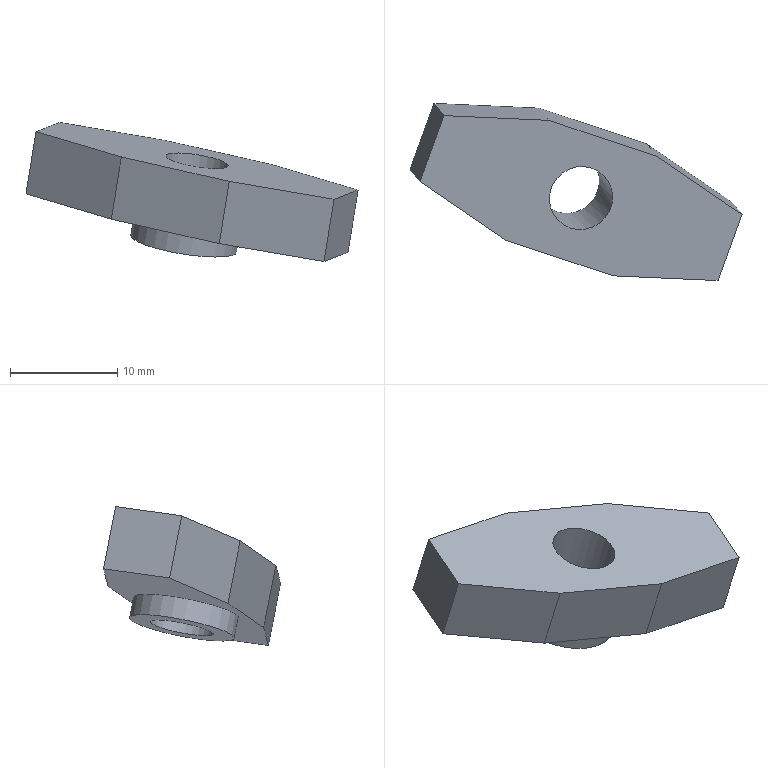Component | NX | MANUAL_NUT | 1 solid | 13 faces | box 31.02 x 16.55 x 12.98 mm | volume 1783 mm3 | plane 11 | cylinder 2 | commonest cylinder face diameters 10 x1 6 x1
STEP:
#1=CARTESIAN_POINT('',(0.,0.,0.));
#2=DIRECTION('',(0.,0.,1.));
#3=DIRECTION('',(1.,0.,0.));
#4=AXIS2_PLACEMENT_3D('',#1,#2,#3);
#5=CARTESIAN_POINT('',(-63.42,-67.809,49.572));
#6=VERTEX_POINT('',#5);
#7=CARTESIAN_POINT('',(-55.446,-73.248,47.215));
#8=VERTEX_POINT('',#7);
#9=CARTESIAN_POINT('',(-63.42,-67.809,49.572));
#10=DIRECTION('',(0.8025,-0.5474,-0.2372));
#11=VECTOR('',#10,1.);
#12=LINE('',#9,#11);
#13=CARTESIAN_POINT('',(-64.357,-66.663,43.757));
#14=DIRECTION('',(-0.5758,-0.8148,-0.06774));
#15=DIRECTION('',(-0.8025,0.5474,0.2372));
#16=AXIS2_PLACEMENT_3D('',#13,#14,#15);
#17=PLANE('',#16);
#18=CARTESIAN_POINT('',(0.,-6.));
#19=DIRECTION('',(-1.,-0.));
#20=VECTOR('',#19,1.);
#21=LINE('',#18,#20);
#22=(GEOMETRIC_REPRESENTATION_CONTEXT(2)PARAMETRIC_REPRESENTATION_CONTEXT()REPRESENTATION_CONTEXT('',''));
#23=DEFINITIONAL_REPRESENTATION('',(#21),#22);
#24=PCURVE('',#17,#23);
#25=CARTESIAN_POINT('',(-70.49,-71.734,49.938));
#26=DIRECTION('',(-0.1562,0.191,-0.9691));
#27=DIRECTION('',(-0.3378,-0.9323,-0.1293));
#28=AXIS2_PLACEMENT_3D('',#25,#26,#27);
#29=PLANE('',#28);
#30=CARTESIAN_POINT('',(-6.,-5.433));
#31=DIRECTION('',(0.2699,-0.9629));
#32=VECTOR('',#31,1.);
#33=LINE('',#30,#32);
#34=(GEOMETRIC_REPRESENTATION_CONTEXT(2)PARAMETRIC_REPRESENTATION_CONTEXT()REPRESENTATION_CONTEXT('',''));
#35=DEFINITIONAL_REPRESENTATION('',(#33),#34);
#36=PCURVE('',#29,#35);
#37=SURFACE_CURVE('',#12,(#24,#36),.PCURVE_S1.);
#38=EDGE_CURVE('',#6,#8,#37,.T.);
#39=ORIENTED_EDGE('',*,*,#38,.T.);
#40=CARTESIAN_POINT('',(-56.384,-72.102,41.4));
#41=VERTEX_POINT('',#40);
#42=CARTESIAN_POINT('',(-56.384,-72.102,41.4));
#43=DIRECTION('',(0.1562,-0.191,0.9691));
#44=VECTOR('',#43,1.);
#45=LINE('',#42,#44);
#46=CARTESIAN_POINT('',(-9.936,0.));
#47=DIRECTION('',(0.,-1.));
#48=VECTOR('',#47,1.);
#49=LINE('',#46,#48);
#50=(GEOMETRIC_REPRESENTATION_CONTEXT(2)PARAMETRIC_REPRESENTATION_CONTEXT()REPRESENTATION_CONTEXT('',''));
#51=DEFINITIONAL_REPRESENTATION('',(#49),#50);
#52=PCURVE('',#17,#51);
#53=CARTESIAN_POINT('',(-57.505,-75.196,40.971));
#54=DIRECTION('',(-0.9282,0.3072,0.2101));
#55=DIRECTION('',(-0.1562,0.191,-0.9691));
#56=AXIS2_PLACEMENT_3D('',#53,#54,#55);
#57=PLANE('',#56);
#58=CARTESIAN_POINT('',(0.,-3.318));
#59=DIRECTION('',(-1.,0.));
#60=VECTOR('',#59,1.);
#61=LINE('',#58,#60);
#62=(GEOMETRIC_REPRESENTATION_CONTEXT(2)PARAMETRIC_REPRESENTATION_CONTEXT()REPRESENTATION_CONTEXT('',''));
#63=DEFINITIONAL_REPRESENTATION('',(#61),#62);
#64=PCURVE('',#57,#63);
#65=SURFACE_CURVE('',#45,(#52,#64),.PCURVE_S1.);
#66=EDGE_CURVE('',#41,#8,#65,.T.);
#67=ORIENTED_EDGE('',*,*,#66,.F.);
#68=CARTESIAN_POINT('',(-64.357,-66.663,43.757));
#69=VERTEX_POINT('',#68);
#70=CARTESIAN_POINT('',(-64.357,-66.663,43.757));
#71=DIRECTION('',(0.8025,-0.5474,-0.2372));
#72=VECTOR('',#71,1.);
#73=LINE('',#70,#72);
#74=CARTESIAN_POINT('',(0.,0.));
#75=DIRECTION('',(-1.,-0.));
#76=VECTOR('',#75,1.);
#77=LINE('',#74,#76);
#78=(GEOMETRIC_REPRESENTATION_CONTEXT(2)PARAMETRIC_REPRESENTATION_CONTEXT()REPRESENTATION_CONTEXT('',''));
#79=DEFINITIONAL_REPRESENTATION('',(#77),#78);
#80=PCURVE('',#17,#79);
#81=CARTESIAN_POINT('',(-71.427,-70.588,44.123));
#82=DIRECTION('',(-0.1562,0.191,-0.9691));
#83=DIRECTION('',(-0.3378,-0.9323,-0.1293));
#84=AXIS2_PLACEMENT_3D('',#81,#82,#83);
#85=PLANE('',#84);
#86=CARTESIAN_POINT('',(-6.,-5.433));
#87=DIRECTION('',(0.2699,-0.9629));
#88=VECTOR('',#87,1.);
#89=LINE('',#86,#88);
#90=(GEOMETRIC_REPRESENTATION_CONTEXT(2)PARAMETRIC_REPRESENTATION_CONTEXT()REPRESENTATION_CONTEXT('',''));
#91=DEFINITIONAL_REPRESENTATION('',(#89),#90);
#92=PCURVE('',#85,#91);
#93=SURFACE_CURVE('',#73,(#80,#92),.PCURVE_S1.);
#94=EDGE_CURVE('',#69,#41,#93,.T.);
#95=ORIENTED_EDGE('',*,*,#94,.F.);
#96=CARTESIAN_POINT('',(-64.357,-66.663,43.757));
#97=DIRECTION('',(0.1562,-0.191,0.9691));
#98=VECTOR('',#97,1.);
#99=LINE('',#96,#98);
#100=CARTESIAN_POINT('',(0.,0.));
#101=DIRECTION('',(0.,-1.));
#102=VECTOR('',#101,1.);
#103=LINE('',#100,#102);
#104=(GEOMETRIC_REPRESENTATION_CONTEXT(2)PARAMETRIC_REPRESENTATION_CONTEXT()REPRESENTATION_CONTEXT('',''));
#105=DEFINITIONAL_REPRESENTATION('',(#103),#104);
#106=PCURVE('',#17,#105);
#107=CARTESIAN_POINT('',(-74.443,-63.325,46.041));
#108=DIRECTION('',(-0.3378,-0.9323,-0.1293));
#109=DIRECTION('',(-0.9282,0.3072,0.2101));
#110=AXIS2_PLACEMENT_3D('',#107,#108,#109);
#111=PLANE('',#110);
#112=CARTESIAN_POINT('',(-10.866,-0.));
#113=DIRECTION('',(0.,-1.));
#114=VECTOR('',#113,1.);
#115=LINE('',#112,#114);
#116=(GEOMETRIC_REPRESENTATION_CONTEXT(2)PARAMETRIC_REPRESENTATION_CONTEXT()REPRESENTATION_CONTEXT('',''));
#117=DEFINITIONAL_REPRESENTATION('',(#115),#116);
#118=PCURVE('',#111,#117);
#119=SURFACE_CURVE('',#99,(#106,#118),.PCURVE_S1.);
#120=EDGE_CURVE('',#69,#6,#119,.T.);
#121=ORIENTED_EDGE('',*,*,#120,.T.);
#122=EDGE_LOOP('',(#39,#67,#95,#121));
#123=FACE_BOUND('',#122,.T.);
#124=ADVANCED_FACE('',(#123),#17,.F.);
#125=CARTESIAN_POINT('',(-57.688,-79.435,46.357));
#126=VERTEX_POINT('',#125);
#127=CARTESIAN_POINT('',(-56.567,-76.341,46.786));
#128=DIRECTION('',(-0.3378,-0.9323,-0.1293));
#129=VECTOR('',#128,1.);
#130=LINE('',#127,#129);
#131=CARTESIAN_POINT('',(-6.,0.));
#132=DIRECTION('',(-0.,1.));
#133=VECTOR('',#132,1.);
#134=LINE('',#131,#133);
#135=(GEOMETRIC_REPRESENTATION_CONTEXT(2)PARAMETRIC_REPRESENTATION_CONTEXT()REPRESENTATION_CONTEXT('',''));
#136=DEFINITIONAL_REPRESENTATION('',(#134),#135);
#137=PCURVE('',#57,#136);
#138=CARTESIAN_POINT('',(0.,-15.));
#139=DIRECTION('',(1.,-0.));
#140=VECTOR('',#139,1.);
#141=LINE('',#138,#140);
#142=(GEOMETRIC_REPRESENTATION_CONTEXT(2)PARAMETRIC_REPRESENTATION_CONTEXT()REPRESENTATION_CONTEXT('',''));
#143=DEFINITIONAL_REPRESENTATION('',(#141),#142);
#144=PCURVE('',#29,#143);
#145=SURFACE_CURVE('',#130,(#137,#144),.PCURVE_S1.);
#146=EDGE_CURVE('',#8,#126,#145,.T.);
#147=ORIENTED_EDGE('',*,*,#146,.T.);
#148=CARTESIAN_POINT('',(-58.625,-78.289,40.542));
#149=VERTEX_POINT('',#148);
#150=CARTESIAN_POINT('',(-58.625,-78.289,40.542));
#151=DIRECTION('',(0.1562,-0.191,0.9691));
#152=VECTOR('',#151,1.);
#153=LINE('',#150,#152);
#154=CARTESIAN_POINT('',(-0.,3.318));
#155=DIRECTION('',(-1.,0.));
#156=VECTOR('',#155,1.);
#157=LINE('',#154,#156);
#158=(GEOMETRIC_REPRESENTATION_CONTEXT(2)PARAMETRIC_REPRESENTATION_CONTEXT()REPRESENTATION_CONTEXT('',''));
#159=DEFINITIONAL_REPRESENTATION('',(#157),#158);
#160=PCURVE('',#57,#159);
#161=CARTESIAN_POINT('',(-58.625,-78.289,40.542));
#162=DIRECTION('',(0.07475,0.9806,0.1812));
#163=DIRECTION('',(0.9849,-0.04414,-0.1674));
#164=AXIS2_PLACEMENT_3D('',#161,#162,#163);
#165=PLANE('',#164);
#166=CARTESIAN_POINT('',(0.,0.));
#167=DIRECTION('',(-0.,-1.));
#168=VECTOR('',#167,1.);
#169=LINE('',#166,#168);
#170=(GEOMETRIC_REPRESENTATION_CONTEXT(2)PARAMETRIC_REPRESENTATION_CONTEXT()REPRESENTATION_CONTEXT('',''));
#171=DEFINITIONAL_REPRESENTATION('',(#169),#170);
#172=PCURVE('',#165,#171);
#173=SURFACE_CURVE('',#153,(#160,#172),.PCURVE_S1.);
#174=EDGE_CURVE('',#149,#126,#173,.T.);
#175=ORIENTED_EDGE('',*,*,#174,.F.);
#176=CARTESIAN_POINT('',(-56.384,-72.102,41.4));
#177=DIRECTION('',(-0.3378,-0.9323,-0.1293));
#178=VECTOR('',#177,1.);
#179=LINE('',#176,#178);
#180=CARTESIAN_POINT('',(0.,-3.318));
#181=DIRECTION('',(-0.,1.));
#182=VECTOR('',#181,1.);
#183=LINE('',#180,#182);
#184=(GEOMETRIC_REPRESENTATION_CONTEXT(2)PARAMETRIC_REPRESENTATION_CONTEXT()REPRESENTATION_CONTEXT('',''));
#185=DEFINITIONAL_REPRESENTATION('',(#183),#184);
#186=PCURVE('',#57,#185);
#187=CARTESIAN_POINT('',(-3.318,-15.));
#188=DIRECTION('',(1.,-0.));
#189=VECTOR('',#188,1.);
#190=LINE('',#187,#189);
#191=(GEOMETRIC_REPRESENTATION_CONTEXT(2)PARAMETRIC_REPRESENTATION_CONTEXT()REPRESENTATION_CONTEXT('',''));
#192=DEFINITIONAL_REPRESENTATION('',(#190),#191);
#193=PCURVE('',#85,#192);
#194=SURFACE_CURVE('',#179,(#186,#193),.PCURVE_S1.);
#195=EDGE_CURVE('',#41,#149,#194,.T.);
#196=ORIENTED_EDGE('',*,*,#195,.F.);
#197=ORIENTED_EDGE('',*,*,#66,.T.);
#198=EDGE_LOOP('',(#147,#175,#196,#197));
#199=FACE_BOUND('',#198,.T.);
#200=ADVANCED_FACE('',(#199),#57,.F.);
#201=CARTESIAN_POINT('',(-67.474,-78.996,48.021));
#202=VERTEX_POINT('',#201);
#203=CARTESIAN_POINT('',(-57.688,-79.435,46.357));
#204=DIRECTION('',(-0.9849,0.04414,0.1674));
#205=VECTOR('',#204,1.);
#206=LINE('',#203,#205);
#207=CARTESIAN_POINT('',(0.,-6.));
#208=DIRECTION('',(-1.,0.));
#209=VECTOR('',#208,1.);
#210=LINE('',#207,#209);
#211=(GEOMETRIC_REPRESENTATION_CONTEXT(2)PARAMETRIC_REPRESENTATION_CONTEXT()REPRESENTATION_CONTEXT('',''));
#212=DEFINITIONAL_REPRESENTATION('',(#210),#211);
#213=PCURVE('',#165,#212);
#214=CARTESIAN_POINT('',(3.318,-15.));
#215=DIRECTION('',(0.2699,0.9629));
#216=VECTOR('',#215,1.);
#217=LINE('',#214,#216);
#218=(GEOMETRIC_REPRESENTATION_CONTEXT(2)PARAMETRIC_REPRESENTATION_CONTEXT()REPRESENTATION_CONTEXT('',''));
#219=DEFINITIONAL_REPRESENTATION('',(#217),#218);
#220=PCURVE('',#29,#219);
#221=SURFACE_CURVE('',#206,(#213,#220),.PCURVE_S1.);
#222=EDGE_CURVE('',#126,#202,#221,.T.);
#223=ORIENTED_EDGE('',*,*,#222,.T.);
#224=CARTESIAN_POINT('',(-68.411,-77.851,42.206));
#225=VERTEX_POINT('',#224);
#226=CARTESIAN_POINT('',(-68.411,-77.851,42.206));
#227=DIRECTION('',(0.1562,-0.191,0.9691));
#228=VECTOR('',#227,1.);
#229=LINE('',#226,#228);
#230=CARTESIAN_POINT('',(-9.936,0.));
#231=DIRECTION('',(-0.,-1.));
#232=VECTOR('',#231,1.);
#233=LINE('',#230,#232);
#234=(GEOMETRIC_REPRESENTATION_CONTEXT(2)PARAMETRIC_REPRESENTATION_CONTEXT()REPRESENTATION_CONTEXT('',''));
#235=DEFINITIONAL_REPRESENTATION('',(#233),#234);
#236=PCURVE('',#165,#235);
#237=CARTESIAN_POINT('',(-73.454,-76.182,43.348));
#238=DIRECTION('',(0.3378,0.9323,0.1293));
#239=DIRECTION('',(0.9282,-0.3072,-0.2101));
#240=AXIS2_PLACEMENT_3D('',#237,#238,#239);
#241=PLANE('',#240);
#242=CARTESIAN_POINT('',(5.433,-0.));
#243=DIRECTION('',(0.,-1.));
#244=VECTOR('',#243,1.);
#245=LINE('',#242,#244);
#246=(GEOMETRIC_REPRESENTATION_CONTEXT(2)PARAMETRIC_REPRESENTATION_CONTEXT()REPRESENTATION_CONTEXT('',''));
#247=DEFINITIONAL_REPRESENTATION('',(#245),#246);
#248=PCURVE('',#241,#247);
#249=SURFACE_CURVE('',#229,(#236,#248),.PCURVE_S1.);
#250=EDGE_CURVE('',#225,#202,#249,.T.);
#251=ORIENTED_EDGE('',*,*,#250,.F.);
#252=CARTESIAN_POINT('',(-58.625,-78.289,40.542));
#253=DIRECTION('',(-0.9849,0.04414,0.1674));
#254=VECTOR('',#253,1.);
#255=LINE('',#252,#254);
#256=CARTESIAN_POINT('',(0.,0.));
#257=DIRECTION('',(-1.,0.));
#258=VECTOR('',#257,1.);
#259=LINE('',#256,#258);
#260=(GEOMETRIC_REPRESENTATION_CONTEXT(2)PARAMETRIC_REPRESENTATION_CONTEXT()REPRESENTATION_CONTEXT('',''));
#261=DEFINITIONAL_REPRESENTATION('',(#259),#260);
#262=PCURVE('',#165,#261);
#263=CARTESIAN_POINT('',(3.318,-15.));
#264=DIRECTION('',(0.2699,0.9629));
#265=VECTOR('',#264,1.);
#266=LINE('',#263,#265);
#267=(GEOMETRIC_REPRESENTATION_CONTEXT(2)PARAMETRIC_REPRESENTATION_CONTEXT()REPRESENTATION_CONTEXT('',''));
#268=DEFINITIONAL_REPRESENTATION('',(#266),#267);
#269=PCURVE('',#85,#268);
#270=SURFACE_CURVE('',#255,(#262,#269),.PCURVE_S1.);
#271=EDGE_CURVE('',#149,#225,#270,.T.);
#272=ORIENTED_EDGE('',*,*,#271,.F.);
#273=ORIENTED_EDGE('',*,*,#174,.T.);
#274=EDGE_LOOP('',(#223,#251,#272,#273));
#275=FACE_BOUND('',#274,.T.);
#276=ADVANCED_FACE('',(#275),#165,.F.);
#277=CARTESIAN_POINT('',(-77.56,-75.658,50.304));
#278=VERTEX_POINT('',#277);
#279=CARTESIAN_POINT('',(-72.517,-77.327,49.162));
#280=DIRECTION('',(-0.9282,0.3072,0.2101));
#281=VECTOR('',#280,1.);
#282=LINE('',#279,#281);
#283=CARTESIAN_POINT('',(0.,-6.));
#284=DIRECTION('',(-1.,0.));
#285=VECTOR('',#284,1.);
#286=LINE('',#283,#285);
#287=(GEOMETRIC_REPRESENTATION_CONTEXT(2)PARAMETRIC_REPRESENTATION_CONTEXT()REPRESENTATION_CONTEXT('',''));
#288=DEFINITIONAL_REPRESENTATION('',(#286),#287);
#289=PCURVE('',#241,#288);
#290=CARTESIAN_POINT('',(6.,-0.));
#291=DIRECTION('',(0.,1.));
#292=VECTOR('',#291,1.);
#293=LINE('',#290,#292);
#294=(GEOMETRIC_REPRESENTATION_CONTEXT(2)PARAMETRIC_REPRESENTATION_CONTEXT()REPRESENTATION_CONTEXT('',''));
#295=DEFINITIONAL_REPRESENTATION('',(#293),#294);
#296=PCURVE('',#29,#295);
#297=SURFACE_CURVE('',#282,(#289,#296),.PCURVE_S1.);
#298=EDGE_CURVE('',#202,#278,#297,.T.);
#299=ORIENTED_EDGE('',*,*,#298,.T.);
#300=CARTESIAN_POINT('',(-78.497,-74.513,44.489));
#301=VERTEX_POINT('',#300);
#302=CARTESIAN_POINT('',(-78.497,-74.513,44.489));
#303=DIRECTION('',(0.1562,-0.191,0.9691));
#304=VECTOR('',#303,1.);
#305=LINE('',#302,#304);
#306=CARTESIAN_POINT('',(-5.433,-0.));
#307=DIRECTION('',(0.,-1.));
#308=VECTOR('',#307,1.);
#309=LINE('',#306,#308);
#310=(GEOMETRIC_REPRESENTATION_CONTEXT(2)PARAMETRIC_REPRESENTATION_CONTEXT()REPRESENTATION_CONTEXT('',''));
#311=DEFINITIONAL_REPRESENTATION('',(#309),#310);
#312=PCURVE('',#241,#311);
#313=CARTESIAN_POINT('',(-78.497,-74.513,44.489));
#314=DIRECTION('',(0.5758,0.8148,0.06774));
#315=DIRECTION('',(0.8025,-0.5474,-0.2372));
#316=AXIS2_PLACEMENT_3D('',#313,#314,#315);
#317=PLANE('',#316);
#318=CARTESIAN_POINT('',(0.,0.));
#319=DIRECTION('',(-0.,-1.));
#320=VECTOR('',#319,1.);
#321=LINE('',#318,#320);
#322=(GEOMETRIC_REPRESENTATION_CONTEXT(2)PARAMETRIC_REPRESENTATION_CONTEXT()REPRESENTATION_CONTEXT('',''));
#323=DEFINITIONAL_REPRESENTATION('',(#321),#322);
#324=PCURVE('',#317,#323);
#325=SURFACE_CURVE('',#305,(#312,#324),.PCURVE_S1.);
#326=EDGE_CURVE('',#301,#278,#325,.T.);
#327=ORIENTED_EDGE('',*,*,#326,.F.);
#328=CARTESIAN_POINT('',(-68.411,-77.851,42.206));
#329=DIRECTION('',(-0.9282,0.3072,0.2101));
#330=VECTOR('',#329,1.);
#331=LINE('',#328,#330);
#332=CARTESIAN_POINT('',(5.433,-0.));
#333=DIRECTION('',(-1.,-0.));
#334=VECTOR('',#333,1.);
#335=LINE('',#332,#334);
#336=(GEOMETRIC_REPRESENTATION_CONTEXT(2)PARAMETRIC_REPRESENTATION_CONTEXT()REPRESENTATION_CONTEXT('',''));
#337=DEFINITIONAL_REPRESENTATION('',(#335),#336);
#338=PCURVE('',#241,#337);
#339=CARTESIAN_POINT('',(6.,-5.433));
#340=DIRECTION('',(-0.,1.));
#341=VECTOR('',#340,1.);
#342=LINE('',#339,#341);
#343=(GEOMETRIC_REPRESENTATION_CONTEXT(2)PARAMETRIC_REPRESENTATION_CONTEXT()REPRESENTATION_CONTEXT('',''));
#344=DEFINITIONAL_REPRESENTATION('',(#342),#343);
#345=PCURVE('',#85,#344);
#346=SURFACE_CURVE('',#331,(#338,#345),.PCURVE_S1.);
#347=EDGE_CURVE('',#225,#301,#346,.T.);
#348=ORIENTED_EDGE('',*,*,#347,.F.);
#349=ORIENTED_EDGE('',*,*,#250,.T.);
#350=EDGE_LOOP('',(#299,#327,#348,#349));
#351=FACE_BOUND('',#350,.T.);
#352=ADVANCED_FACE('',(#351),#241,.F.);
#353=CARTESIAN_POINT('',(-85.533,-70.219,52.661));
#354=VERTEX_POINT('',#353);
#355=CARTESIAN_POINT('',(-77.56,-75.658,50.304));
#356=DIRECTION('',(-0.8025,0.5474,0.2372));
#357=VECTOR('',#356,1.);
#358=LINE('',#355,#357);
#359=CARTESIAN_POINT('',(0.,-6.));
#360=DIRECTION('',(-1.,0.));
#361=VECTOR('',#360,1.);
#362=LINE('',#359,#361);
#363=(GEOMETRIC_REPRESENTATION_CONTEXT(2)PARAMETRIC_REPRESENTATION_CONTEXT()REPRESENTATION_CONTEXT('',''));
#364=DEFINITIONAL_REPRESENTATION('',(#362),#363);
#365=PCURVE('',#317,#364);
#366=CARTESIAN_POINT('',(6.,5.433));
#367=DIRECTION('',(-0.2699,0.9629));
#368=VECTOR('',#367,1.);
#369=LINE('',#366,#368);
#370=(GEOMETRIC_REPRESENTATION_CONTEXT(2)PARAMETRIC_REPRESENTATION_CONTEXT()REPRESENTATION_CONTEXT('',''));
#371=DEFINITIONAL_REPRESENTATION('',(#369),#370);
#372=PCURVE('',#29,#371);
#373=SURFACE_CURVE('',#358,(#365,#372),.PCURVE_S1.);
#374=EDGE_CURVE('',#278,#354,#373,.T.);
#375=ORIENTED_EDGE('',*,*,#374,.T.);
#376=CARTESIAN_POINT('',(-86.47,-69.073,46.846));
#377=VERTEX_POINT('',#376);
#378=CARTESIAN_POINT('',(-86.47,-69.073,46.846));
#379=DIRECTION('',(0.1562,-0.191,0.9691));
#380=VECTOR('',#379,1.);
#381=LINE('',#378,#380);
#382=CARTESIAN_POINT('',(-9.936,-0.));
#383=DIRECTION('',(-0.,-1.));
#384=VECTOR('',#383,1.);
#385=LINE('',#382,#384);
#386=(GEOMETRIC_REPRESENTATION_CONTEXT(2)PARAMETRIC_REPRESENTATION_CONTEXT()REPRESENTATION_CONTEXT('',''));
#387=DEFINITIONAL_REPRESENTATION('',(#385),#386);
#388=PCURVE('',#317,#387);
#389=CARTESIAN_POINT('',(-85.349,-65.98,47.275));
#390=DIRECTION('',(0.9282,-0.3072,-0.2101));
#391=DIRECTION('',(0.1562,-0.191,0.9691));
#392=AXIS2_PLACEMENT_3D('',#389,#390,#391);
#393=PLANE('',#392);
#394=CARTESIAN_POINT('',(0.,3.318));
#395=DIRECTION('',(1.,0.));
#396=VECTOR('',#395,1.);
#397=LINE('',#394,#396);
#398=(GEOMETRIC_REPRESENTATION_CONTEXT(2)PARAMETRIC_REPRESENTATION_CONTEXT()REPRESENTATION_CONTEXT('',''));
#399=DEFINITIONAL_REPRESENTATION('',(#397),#398);
#400=PCURVE('',#393,#399);
#401=SURFACE_CURVE('',#381,(#388,#400),.PCURVE_S1.);
#402=EDGE_CURVE('',#377,#354,#401,.T.);
#403=ORIENTED_EDGE('',*,*,#402,.F.);
#404=CARTESIAN_POINT('',(-78.497,-74.513,44.489));
#405=DIRECTION('',(-0.8025,0.5474,0.2372));
#406=VECTOR('',#405,1.);
#407=LINE('',#404,#406);
#408=CARTESIAN_POINT('',(0.,0.));
#409=DIRECTION('',(-1.,0.));
#410=VECTOR('',#409,1.);
#411=LINE('',#408,#410);
#412=(GEOMETRIC_REPRESENTATION_CONTEXT(2)PARAMETRIC_REPRESENTATION_CONTEXT()REPRESENTATION_CONTEXT('',''));
#413=DEFINITIONAL_REPRESENTATION('',(#411),#412);
#414=PCURVE('',#317,#413);
#415=CARTESIAN_POINT('',(6.,5.433));
#416=DIRECTION('',(-0.2699,0.9629));
#417=VECTOR('',#416,1.);
#418=LINE('',#415,#417);
#419=(GEOMETRIC_REPRESENTATION_CONTEXT(2)PARAMETRIC_REPRESENTATION_CONTEXT()REPRESENTATION_CONTEXT('',''));
#420=DEFINITIONAL_REPRESENTATION('',(#418),#419);
#421=PCURVE('',#85,#420);
#422=SURFACE_CURVE('',#407,(#414,#421),.PCURVE_S1.);
#423=EDGE_CURVE('',#301,#377,#422,.T.);
#424=ORIENTED_EDGE('',*,*,#423,.F.);
#425=ORIENTED_EDGE('',*,*,#326,.T.);
#426=EDGE_LOOP('',(#375,#403,#424,#425));
#427=FACE_BOUND('',#426,.T.);
#428=ADVANCED_FACE('',(#427),#317,.F.);
#429=CARTESIAN_POINT('',(-83.291,-64.032,53.519));
#430=VERTEX_POINT('',#429);
#431=CARTESIAN_POINT('',(-84.412,-67.126,53.09));
#432=DIRECTION('',(0.3378,0.9323,0.1293));
#433=VECTOR('',#432,1.);
#434=LINE('',#431,#433);
#435=CARTESIAN_POINT('',(6.,-0.));
#436=DIRECTION('',(-0.,-1.));
#437=VECTOR('',#436,1.);
#438=LINE('',#435,#437);
#439=(GEOMETRIC_REPRESENTATION_CONTEXT(2)PARAMETRIC_REPRESENTATION_CONTEXT()REPRESENTATION_CONTEXT('',''));
#440=DEFINITIONAL_REPRESENTATION('',(#438),#439);
#441=PCURVE('',#393,#440);
#442=CARTESIAN_POINT('',(-0.,15.));
#443=DIRECTION('',(-1.,0.));
#444=VECTOR('',#443,1.);
#445=LINE('',#442,#444);
#446=(GEOMETRIC_REPRESENTATION_CONTEXT(2)PARAMETRIC_REPRESENTATION_CONTEXT()REPRESENTATION_CONTEXT('',''));
#447=DEFINITIONAL_REPRESENTATION('',(#445),#446);
#448=PCURVE('',#29,#447);
#449=SURFACE_CURVE('',#434,(#441,#448),.PCURVE_S1.);
#450=EDGE_CURVE('',#354,#430,#449,.T.);
#451=ORIENTED_EDGE('',*,*,#450,.T.);
#452=CARTESIAN_POINT('',(-84.228,-62.886,47.704));
#453=VERTEX_POINT('',#452);
#454=CARTESIAN_POINT('',(-84.228,-62.886,47.704));
#455=DIRECTION('',(0.1562,-0.191,0.9691));
#456=VECTOR('',#455,1.);
#457=LINE('',#454,#456);
#458=CARTESIAN_POINT('',(0.,-3.318));
#459=DIRECTION('',(1.,0.));
#460=VECTOR('',#459,1.);
#461=LINE('',#458,#460);
#462=(GEOMETRIC_REPRESENTATION_CONTEXT(2)PARAMETRIC_REPRESENTATION_CONTEXT()REPRESENTATION_CONTEXT('',''));
#463=DEFINITIONAL_REPRESENTATION('',(#461),#462);
#464=PCURVE('',#393,#463);
#465=CARTESIAN_POINT('',(-84.228,-62.886,47.704));
#466=DIRECTION('',(-0.07475,-0.9806,-0.1812));
#467=DIRECTION('',(-0.9849,0.04414,0.1674));
#468=AXIS2_PLACEMENT_3D('',#465,#466,#467);
#469=PLANE('',#468);
#470=CARTESIAN_POINT('',(0.,0.));
#471=DIRECTION('',(0.,-1.));
#472=VECTOR('',#471,1.);
#473=LINE('',#470,#472);
#474=(GEOMETRIC_REPRESENTATION_CONTEXT(2)PARAMETRIC_REPRESENTATION_CONTEXT()REPRESENTATION_CONTEXT('',''));
#475=DEFINITIONAL_REPRESENTATION('',(#473),#474);
#476=PCURVE('',#469,#475);
#477=SURFACE_CURVE('',#457,(#464,#476),.PCURVE_S1.);
#478=EDGE_CURVE('',#453,#430,#477,.T.);
#479=ORIENTED_EDGE('',*,*,#478,.F.);
#480=CARTESIAN_POINT('',(-86.47,-69.073,46.846));
#481=DIRECTION('',(0.3378,0.9323,0.1293));
#482=VECTOR('',#481,1.);
#483=LINE('',#480,#482);
#484=CARTESIAN_POINT('',(0.,3.318));
#485=DIRECTION('',(-0.,-1.));
#486=VECTOR('',#485,1.);
#487=LINE('',#484,#486);
#488=(GEOMETRIC_REPRESENTATION_CONTEXT(2)PARAMETRIC_REPRESENTATION_CONTEXT()REPRESENTATION_CONTEXT('',''));
#489=DEFINITIONAL_REPRESENTATION('',(#487),#488);
#490=PCURVE('',#393,#489);
#491=CARTESIAN_POINT('',(3.318,15.));
#492=DIRECTION('',(-1.,0.));
#493=VECTOR('',#492,1.);
#494=LINE('',#491,#493);
#495=(GEOMETRIC_REPRESENTATION_CONTEXT(2)PARAMETRIC_REPRESENTATION_CONTEXT()REPRESENTATION_CONTEXT('',''));
#496=DEFINITIONAL_REPRESENTATION('',(#494),#495);
#497=PCURVE('',#85,#496);
#498=SURFACE_CURVE('',#483,(#490,#497),.PCURVE_S1.);
#499=EDGE_CURVE('',#377,#453,#498,.T.);
#500=ORIENTED_EDGE('',*,*,#499,.F.);
#501=ORIENTED_EDGE('',*,*,#402,.T.);
#502=EDGE_LOOP('',(#451,#479,#500,#501));
#503=FACE_BOUND('',#502,.T.);
#504=ADVANCED_FACE('',(#503),#393,.F.);
#505=CARTESIAN_POINT('',(-73.506,-64.471,51.855));
#506=VERTEX_POINT('',#505);
#507=CARTESIAN_POINT('',(-83.291,-64.032,53.519));
#508=DIRECTION('',(0.9849,-0.04414,-0.1674));
#509=VECTOR('',#508,1.);
#510=LINE('',#507,#509);
#511=CARTESIAN_POINT('',(-0.,-6.));
#512=DIRECTION('',(-1.,-0.));
#513=VECTOR('',#512,1.);
#514=LINE('',#511,#513);
#515=(GEOMETRIC_REPRESENTATION_CONTEXT(2)PARAMETRIC_REPRESENTATION_CONTEXT()REPRESENTATION_CONTEXT('',''));
#516=DEFINITIONAL_REPRESENTATION('',(#514),#515);
#517=PCURVE('',#469,#516);
#518=CARTESIAN_POINT('',(-3.318,15.));
#519=DIRECTION('',(-0.2699,-0.9629));
#520=VECTOR('',#519,1.);
#521=LINE('',#518,#520);
#522=(GEOMETRIC_REPRESENTATION_CONTEXT(2)PARAMETRIC_REPRESENTATION_CONTEXT()REPRESENTATION_CONTEXT('',''));
#523=DEFINITIONAL_REPRESENTATION('',(#521),#522);
#524=PCURVE('',#29,#523);
#525=SURFACE_CURVE('',#510,(#517,#524),.PCURVE_S1.);
#526=EDGE_CURVE('',#430,#506,#525,.T.);
#527=ORIENTED_EDGE('',*,*,#526,.T.);
#528=CARTESIAN_POINT('',(-74.443,-63.325,46.041));
#529=VERTEX_POINT('',#528);
#530=CARTESIAN_POINT('',(-74.443,-63.325,46.041));
#531=DIRECTION('',(0.1562,-0.191,0.9691));
#532=VECTOR('',#531,1.);
#533=LINE('',#530,#532);
#534=CARTESIAN_POINT('',(-9.936,0.));
#535=DIRECTION('',(0.,-1.));
#536=VECTOR('',#535,1.);
#537=LINE('',#534,#536);
#538=(GEOMETRIC_REPRESENTATION_CONTEXT(2)PARAMETRIC_REPRESENTATION_CONTEXT()REPRESENTATION_CONTEXT('',''));
#539=DEFINITIONAL_REPRESENTATION('',(#537),#538);
#540=PCURVE('',#469,#539);
#541=CARTESIAN_POINT('',(0.,0.));
#542=DIRECTION('',(0.,-1.));
#543=VECTOR('',#542,1.);
#544=LINE('',#541,#543);
#545=(GEOMETRIC_REPRESENTATION_CONTEXT(2)PARAMETRIC_REPRESENTATION_CONTEXT()REPRESENTATION_CONTEXT('',''));
#546=DEFINITIONAL_REPRESENTATION('',(#544),#545);
#547=PCURVE('',#111,#546);
#548=SURFACE_CURVE('',#533,(#540,#547),.PCURVE_S1.);
#549=EDGE_CURVE('',#529,#506,#548,.T.);
#550=ORIENTED_EDGE('',*,*,#549,.F.);
#551=CARTESIAN_POINT('',(-84.228,-62.886,47.704));
#552=DIRECTION('',(0.9849,-0.04414,-0.1674));
#553=VECTOR('',#552,1.);
#554=LINE('',#551,#553);
#555=CARTESIAN_POINT('',(0.,0.));
#556=DIRECTION('',(-1.,-0.));
#557=VECTOR('',#556,1.);
#558=LINE('',#555,#557);
#559=(GEOMETRIC_REPRESENTATION_CONTEXT(2)PARAMETRIC_REPRESENTATION_CONTEXT()REPRESENTATION_CONTEXT('',''));
#560=DEFINITIONAL_REPRESENTATION('',(#558),#559);
#561=PCURVE('',#469,#560);
#562=CARTESIAN_POINT('',(-3.318,15.));
#563=DIRECTION('',(-0.2699,-0.9629));
#564=VECTOR('',#563,1.);
#565=LINE('',#562,#564);
#566=(GEOMETRIC_REPRESENTATION_CONTEXT(2)PARAMETRIC_REPRESENTATION_CONTEXT()REPRESENTATION_CONTEXT('',''));
#567=DEFINITIONAL_REPRESENTATION('',(#565),#566);
#568=PCURVE('',#85,#567);
#569=SURFACE_CURVE('',#554,(#561,#568),.PCURVE_S1.);
#570=EDGE_CURVE('',#453,#529,#569,.T.);
#571=ORIENTED_EDGE('',*,*,#570,.F.);
#572=ORIENTED_EDGE('',*,*,#478,.T.);
#573=EDGE_LOOP('',(#527,#550,#571,#572));
#574=FACE_BOUND('',#573,.T.);
#575=ADVANCED_FACE('',(#574),#469,.F.);
#576=CARTESIAN_POINT('',(-73.506,-64.471,51.855));
#577=DIRECTION('',(0.9282,-0.3072,-0.2101));
#578=VECTOR('',#577,1.);
#579=LINE('',#576,#578);
#580=CARTESIAN_POINT('',(0.,-6.));
#581=DIRECTION('',(-1.,0.));
#582=VECTOR('',#581,1.);
#583=LINE('',#580,#582);
#584=(GEOMETRIC_REPRESENTATION_CONTEXT(2)PARAMETRIC_REPRESENTATION_CONTEXT()REPRESENTATION_CONTEXT('',''));
#585=DEFINITIONAL_REPRESENTATION('',(#583),#584);
#586=PCURVE('',#111,#585);
#587=CARTESIAN_POINT('',(-6.,5.433));
#588=DIRECTION('',(0.,-1.));
#589=VECTOR('',#588,1.);
#590=LINE('',#587,#589);
#591=(GEOMETRIC_REPRESENTATION_CONTEXT(2)PARAMETRIC_REPRESENTATION_CONTEXT()REPRESENTATION_CONTEXT('',''));
#592=DEFINITIONAL_REPRESENTATION('',(#590),#591);
#593=PCURVE('',#29,#592);
#594=SURFACE_CURVE('',#579,(#586,#593),.PCURVE_S1.);
#595=EDGE_CURVE('',#506,#6,#594,.T.);
#596=ORIENTED_EDGE('',*,*,#595,.T.);
#597=ORIENTED_EDGE('',*,*,#120,.F.);
#598=CARTESIAN_POINT('',(-69.4,-64.994,44.899));
#599=DIRECTION('',(0.9282,-0.3072,-0.2101));
#600=VECTOR('',#599,1.);
#601=LINE('',#598,#600);
#602=CARTESIAN_POINT('',(-5.433,0.));
#603=DIRECTION('',(-1.,-0.));
#604=VECTOR('',#603,1.);
#605=LINE('',#602,#604);
#606=(GEOMETRIC_REPRESENTATION_CONTEXT(2)PARAMETRIC_REPRESENTATION_CONTEXT()REPRESENTATION_CONTEXT('',''));
#607=DEFINITIONAL_REPRESENTATION('',(#605),#606);
#608=PCURVE('',#111,#607);
#609=CARTESIAN_POINT('',(-6.,-0.));
#610=DIRECTION('',(-0.,-1.));
#611=VECTOR('',#610,1.);
#612=LINE('',#609,#611);
#613=(GEOMETRIC_REPRESENTATION_CONTEXT(2)PARAMETRIC_REPRESENTATION_CONTEXT()REPRESENTATION_CONTEXT('',''));
#614=DEFINITIONAL_REPRESENTATION('',(#612),#613);
#615=PCURVE('',#85,#614);
#616=SURFACE_CURVE('',#601,(#608,#615),.PCURVE_S1.);
#617=EDGE_CURVE('',#529,#69,#616,.T.);
#618=ORIENTED_EDGE('',*,*,#617,.F.);
#619=ORIENTED_EDGE('',*,*,#549,.T.);
#620=EDGE_LOOP('',(#596,#597,#618,#619));
#621=FACE_BOUND('',#620,.T.);
#622=ADVANCED_FACE('',(#621),#111,.F.);
#623=CARTESIAN_POINT('',(-73.116,-75.249,43.477));
#624=VERTEX_POINT('',#623);
#625=CARTESIAN_POINT('',(-71.427,-70.588,44.123));
#626=DIRECTION('',(-0.1562,0.191,-0.9691));
#627=DIRECTION('',(-0.3378,-0.9323,-0.1293));
#628=AXIS2_PLACEMENT_3D('',#625,#626,#627);
#629=CIRCLE('',#628,5.);
#630=CARTESIAN_POINT('',(0.,0.));
#631=DIRECTION('',(1.,0.));
#632=AXIS2_PLACEMENT_2D('',#630,#631);
#633=CIRCLE('',#632,5.);
#634=(GEOMETRIC_REPRESENTATION_CONTEXT(2)PARAMETRIC_REPRESENTATION_CONTEXT()REPRESENTATION_CONTEXT('',''));
#635=DEFINITIONAL_REPRESENTATION('',(#633),#634);
#636=PCURVE('',#85,#635);
#637=CARTESIAN_POINT('',(-71.739,-70.206,42.185));
#638=DIRECTION('',(0.1562,-0.191,0.9691));
#639=DIRECTION('',(0.3378,0.9323,0.1293));
#640=AXIS2_PLACEMENT_3D('',#637,#638,#639);
#641=CYLINDRICAL_SURFACE('',#640,5.);
#642=CARTESIAN_POINT('',(9.425,2.));
#643=DIRECTION('',(-1.,0.));
#644=VECTOR('',#643,1.);
#645=LINE('',#642,#644);
#646=(GEOMETRIC_REPRESENTATION_CONTEXT(2)PARAMETRIC_REPRESENTATION_CONTEXT()REPRESENTATION_CONTEXT('',''));
#647=DEFINITIONAL_REPRESENTATION('',(#645),#646);
#648=PCURVE('',#641,#647);
#649=SURFACE_CURVE('',#629,(#636,#648),.PCURVE_S1.);
#650=EDGE_CURVE('',#624,#624,#649,.T.);
#651=ORIENTED_EDGE('',*,*,#650,.F.);
#652=EDGE_LOOP('',(#651));
#653=FACE_BOUND('',#652,.T.);
#654=ORIENTED_EDGE('',*,*,#617,.T.);
#655=ORIENTED_EDGE('',*,*,#94,.T.);
#656=ORIENTED_EDGE('',*,*,#195,.T.);
#657=ORIENTED_EDGE('',*,*,#271,.T.);
#658=ORIENTED_EDGE('',*,*,#347,.T.);
#659=ORIENTED_EDGE('',*,*,#423,.T.);
#660=ORIENTED_EDGE('',*,*,#499,.T.);
#661=ORIENTED_EDGE('',*,*,#570,.T.);
#662=EDGE_LOOP('',(#654,#655,#656,#657,#658,#659,#660,#661));
#663=FACE_BOUND('',#662,.T.);
#664=ADVANCED_FACE('',(#653,#663),#85,.T.);
#665=CARTESIAN_POINT('',(-71.503,-74.53,49.55));
#666=VERTEX_POINT('',#665);
#667=CARTESIAN_POINT('',(-70.49,-71.734,49.938));
#668=DIRECTION('',(-0.1562,0.191,-0.9691));
#669=DIRECTION('',(-0.3378,-0.9323,-0.1293));
#670=AXIS2_PLACEMENT_3D('',#667,#668,#669);
#671=CIRCLE('',#670,3.);
#672=CARTESIAN_POINT('',(0.,0.));
#673=DIRECTION('',(1.,0.));
#674=AXIS2_PLACEMENT_2D('',#672,#673);
#675=CIRCLE('',#674,3.);
#676=(GEOMETRIC_REPRESENTATION_CONTEXT(2)PARAMETRIC_REPRESENTATION_CONTEXT()REPRESENTATION_CONTEXT('',''));
#677=DEFINITIONAL_REPRESENTATION('',(#675),#676);
#678=PCURVE('',#29,#677);
#679=CARTESIAN_POINT('',(-68.615,-74.025,61.567));
#680=DIRECTION('',(-0.1562,0.191,-0.9691));
#681=DIRECTION('',(-0.3378,-0.9323,-0.1293));
#682=AXIS2_PLACEMENT_3D('',#679,#680,#681);
#683=CYLINDRICAL_SURFACE('',#682,3.);
#684=CARTESIAN_POINT('',(0.,12.));
#685=DIRECTION('',(1.,0.));
#686=VECTOR('',#685,1.);
#687=LINE('',#684,#686);
#688=(GEOMETRIC_REPRESENTATION_CONTEXT(2)PARAMETRIC_REPRESENTATION_CONTEXT()REPRESENTATION_CONTEXT('',''));
#689=DEFINITIONAL_REPRESENTATION('',(#687),#688);
#690=PCURVE('',#683,#689);
#691=SURFACE_CURVE('',#671,(#678,#690),.PCURVE_S1.);
#692=EDGE_CURVE('',#666,#666,#691,.T.);
#693=ORIENTED_EDGE('',*,*,#692,.T.);
#694=EDGE_LOOP('',(#693));
#695=FACE_BOUND('',#694,.T.);
#696=ORIENTED_EDGE('',*,*,#38,.F.);
#697=ORIENTED_EDGE('',*,*,#595,.F.);
#698=ORIENTED_EDGE('',*,*,#526,.F.);
#699=ORIENTED_EDGE('',*,*,#450,.F.);
#700=ORIENTED_EDGE('',*,*,#374,.F.);
#701=ORIENTED_EDGE('',*,*,#298,.F.);
#702=ORIENTED_EDGE('',*,*,#222,.F.);
#703=ORIENTED_EDGE('',*,*,#146,.F.);
#704=EDGE_LOOP('',(#696,#697,#698,#699,#700,#701,#702,#703));
#705=FACE_BOUND('',#704,.T.);
#706=ADVANCED_FACE('',(#695,#705),#29,.F.);
#707=CARTESIAN_POINT('',(-73.428,-74.867,41.539));
#708=VERTEX_POINT('',#707);
#709=CARTESIAN_POINT('',(-71.739,-70.206,42.185));
#710=DIRECTION('',(-0.1562,0.191,-0.9691));
#711=DIRECTION('',(-0.3378,-0.9323,-0.1293));
#712=AXIS2_PLACEMENT_3D('',#709,#710,#711);
#713=CIRCLE('',#712,5.);
#714=CARTESIAN_POINT('',(9.425,0.));
#715=DIRECTION('',(-1.,0.));
#716=VECTOR('',#715,1.);
#717=LINE('',#714,#716);
#718=(GEOMETRIC_REPRESENTATION_CONTEXT(2)PARAMETRIC_REPRESENTATION_CONTEXT()REPRESENTATION_CONTEXT('',''));
#719=DEFINITIONAL_REPRESENTATION('',(#717),#718);
#720=PCURVE('',#641,#719);
#721=CARTESIAN_POINT('',(-71.739,-70.206,42.185));
#722=DIRECTION('',(-0.1562,0.191,-0.9691));
#723=DIRECTION('',(-0.3378,-0.9323,-0.1293));
#724=AXIS2_PLACEMENT_3D('',#721,#722,#723);
#725=PLANE('',#724);
#726=CARTESIAN_POINT('',(0.,0.));
#727=DIRECTION('',(1.,0.));
#728=AXIS2_PLACEMENT_2D('',#726,#727);
#729=CIRCLE('',#728,5.);
#730=(GEOMETRIC_REPRESENTATION_CONTEXT(2)PARAMETRIC_REPRESENTATION_CONTEXT()REPRESENTATION_CONTEXT('',''));
#731=DEFINITIONAL_REPRESENTATION('',(#729),#730);
#732=PCURVE('',#725,#731);
#733=SURFACE_CURVE('',#713,(#720,#732),.PCURVE_S1.);
#734=EDGE_CURVE('',#708,#708,#733,.T.);
#735=ORIENTED_EDGE('',*,*,#734,.F.);
#736=CARTESIAN_POINT('',(-73.428,-74.867,41.539));
#737=CARTESIAN_POINT('',(-73.116,-75.249,43.477));
#738=B_SPLINE_CURVE_WITH_KNOTS('',1,(#736,#737),.UNSPECIFIED.,.F.,.F.,(2,2),(0.,2.),.PIECEWISE_BEZIER_KNOTS.);
#739=CARTESIAN_POINT('',(9.425,0.));
#740=DIRECTION('',(0.,1.));
#741=VECTOR('',#740,1.);
#742=LINE('',#739,#741);
#743=(GEOMETRIC_REPRESENTATION_CONTEXT(2)PARAMETRIC_REPRESENTATION_CONTEXT()REPRESENTATION_CONTEXT('',''));
#744=DEFINITIONAL_REPRESENTATION('',(#742),#743);
#745=PCURVE('',#641,#744);
#746=CARTESIAN_POINT('',(3.142,0.));
#747=DIRECTION('',(0.,1.));
#748=VECTOR('',#747,1.);
#749=LINE('',#746,#748);
#750=(GEOMETRIC_REPRESENTATION_CONTEXT(2)PARAMETRIC_REPRESENTATION_CONTEXT()REPRESENTATION_CONTEXT('',''));
#751=DEFINITIONAL_REPRESENTATION('',(#749),#750);
#752=PCURVE('',#641,#751);
#753=SEAM_CURVE('',#738,(#745,#752),.PCURVE_S1.);
#754=EDGE_CURVE('',#708,#624,#753,.T.);
#755=ORIENTED_EDGE('',*,*,#754,.T.);
#756=ORIENTED_EDGE('',*,*,#650,.T.);
#757=ORIENTED_EDGE('',*,*,#754,.F.);
#758=EDGE_LOOP('',(#735,#755,#756,#757));
#759=FACE_BOUND('',#758,.T.);
#760=ADVANCED_FACE('',(#759),#641,.T.);
#761=CARTESIAN_POINT('',(-68.955,-71.127,41.555));
#762=VERTEX_POINT('',#761);
#763=CARTESIAN_POINT('',(-72.753,-73.003,41.797));
#764=VERTEX_POINT('',#763);
#765=CARTESIAN_POINT('',(-71.739,-70.206,42.185));
#766=DIRECTION('',(-0.1562,0.191,-0.9691));
#767=DIRECTION('',(0.9282,-0.3072,-0.2101));
#768=AXIS2_PLACEMENT_3D('',#765,#766,#767);
#769=CIRCLE('',#768,3.);
#770=CARTESIAN_POINT('',(0.,0.));
#771=DIRECTION('',(-0.,-1.));
#772=AXIS2_PLACEMENT_2D('',#770,#771);
#773=CIRCLE('',#772,3.);
#774=(GEOMETRIC_REPRESENTATION_CONTEXT(2)PARAMETRIC_REPRESENTATION_CONTEXT()REPRESENTATION_CONTEXT('',''));
#775=DEFINITIONAL_REPRESENTATION('',(#773),#774);
#776=PCURVE('',#725,#775);
#777=CARTESIAN_POINT('',(4.712,20.));
#778=DIRECTION('',(1.,0.));
#779=VECTOR('',#778,1.);
#780=LINE('',#777,#779);
#781=(GEOMETRIC_REPRESENTATION_CONTEXT(2)PARAMETRIC_REPRESENTATION_CONTEXT()REPRESENTATION_CONTEXT('',''));
#782=DEFINITIONAL_REPRESENTATION('',(#780),#781);
#783=PCURVE('',#683,#782);
#784=SURFACE_CURVE('',#769,(#776,#783),.PCURVE_S1.);
#785=EDGE_CURVE('',#762,#764,#784,.T.);
#786=ORIENTED_EDGE('',*,*,#785,.F.);
#787=CARTESIAN_POINT('',(-71.739,-70.206,42.185));
#788=DIRECTION('',(-0.1562,0.191,-0.9691));
#789=DIRECTION('',(0.9282,-0.3072,-0.2101));
#790=AXIS2_PLACEMENT_3D('',#787,#788,#789);
#791=CIRCLE('',#790,3.);
#792=CARTESIAN_POINT('',(0.,0.));
#793=DIRECTION('',(-0.,-1.));
#794=AXIS2_PLACEMENT_2D('',#792,#793);
#795=CIRCLE('',#794,3.);
#796=(GEOMETRIC_REPRESENTATION_CONTEXT(2)PARAMETRIC_REPRESENTATION_CONTEXT()REPRESENTATION_CONTEXT('',''));
#797=DEFINITIONAL_REPRESENTATION('',(#795),#796);
#798=PCURVE('',#725,#797);
#799=CARTESIAN_POINT('',(-1.571,20.));
#800=DIRECTION('',(1.,0.));
#801=VECTOR('',#800,1.);
#802=LINE('',#799,#801);
#803=(GEOMETRIC_REPRESENTATION_CONTEXT(2)PARAMETRIC_REPRESENTATION_CONTEXT()REPRESENTATION_CONTEXT('',''));
#804=DEFINITIONAL_REPRESENTATION('',(#802),#803);
#805=PCURVE('',#683,#804);
#806=SURFACE_CURVE('',#791,(#798,#805),.PCURVE_S1.);
#807=EDGE_CURVE('',#764,#762,#806,.T.);
#808=ORIENTED_EDGE('',*,*,#807,.F.);
#809=EDGE_LOOP('',(#786,#808));
#810=FACE_BOUND('',#809,.T.);
#811=ORIENTED_EDGE('',*,*,#734,.T.);
#812=EDGE_LOOP('',(#811));
#813=FACE_BOUND('',#812,.T.);
#814=ADVANCED_FACE('',(#810,#813),#725,.T.);
#815=ORIENTED_EDGE('',*,*,#807,.F.);
#816=CARTESIAN_POINT('',(-71.503,-74.53,49.55));
#817=CARTESIAN_POINT('',(-72.753,-73.003,41.797));
#818=B_SPLINE_CURVE_WITH_KNOTS('',1,(#816,#817),.UNSPECIFIED.,.F.,.F.,(2,2),(12.,20.),.PIECEWISE_BEZIER_KNOTS.);
#819=CARTESIAN_POINT('',(0.,0.));
#820=DIRECTION('',(0.,1.));
#821=VECTOR('',#820,1.);
#822=LINE('',#819,#821);
#823=(GEOMETRIC_REPRESENTATION_CONTEXT(2)PARAMETRIC_REPRESENTATION_CONTEXT()REPRESENTATION_CONTEXT('',''));
#824=DEFINITIONAL_REPRESENTATION('',(#822),#823);
#825=PCURVE('',#683,#824);
#826=CARTESIAN_POINT('',(6.283,0.));
#827=DIRECTION('',(0.,1.));
#828=VECTOR('',#827,1.);
#829=LINE('',#826,#828);
#830=(GEOMETRIC_REPRESENTATION_CONTEXT(2)PARAMETRIC_REPRESENTATION_CONTEXT()REPRESENTATION_CONTEXT('',''));
#831=DEFINITIONAL_REPRESENTATION('',(#829),#830);
#832=PCURVE('',#683,#831);
#833=SEAM_CURVE('',#818,(#825,#832),.PCURVE_S1.);
#834=EDGE_CURVE('',#666,#764,#833,.T.);
#835=ORIENTED_EDGE('',*,*,#834,.F.);
#836=ORIENTED_EDGE('',*,*,#692,.T.);
#837=ORIENTED_EDGE('',*,*,#834,.T.);
#838=ORIENTED_EDGE('',*,*,#785,.F.);
#839=EDGE_LOOP('',(#815,#835,#836,#837,#838));
#840=FACE_BOUND('',#839,.F.);
#841=ADVANCED_FACE('',(#840),#683,.F.);
#842=CLOSED_SHELL('',(#124,#200,#276,#352,#428,#504,#575,#622,#664,#706,#760,#814,#841));
#843=MANIFOLD_SOLID_BREP('',#842);
#844=(LENGTH_UNIT()NAMED_UNIT(*)SI_UNIT(.MILLI.,.METRE.));
#845=UNCERTAINTY_MEASURE_WITH_UNIT(LENGTH_MEASURE(0.000002),#844,'','');
#846=(NAMED_UNIT(*)PLANE_ANGLE_UNIT()SI_UNIT($,.RADIAN.));
#847=(NAMED_UNIT(*)SI_UNIT($,.STERADIAN.)SOLID_ANGLE_UNIT());
#848=(GEOMETRIC_REPRESENTATION_CONTEXT(3)GLOBAL_UNCERTAINTY_ASSIGNED_CONTEXT((#845))GLOBAL_UNIT_ASSIGNED_CONTEXT((#844,#846,#847))REPRESENTATION_CONTEXT('',''));
#849=ADVANCED_BREP_SHAPE_REPRESENTATION('',(#4,#843),#848);